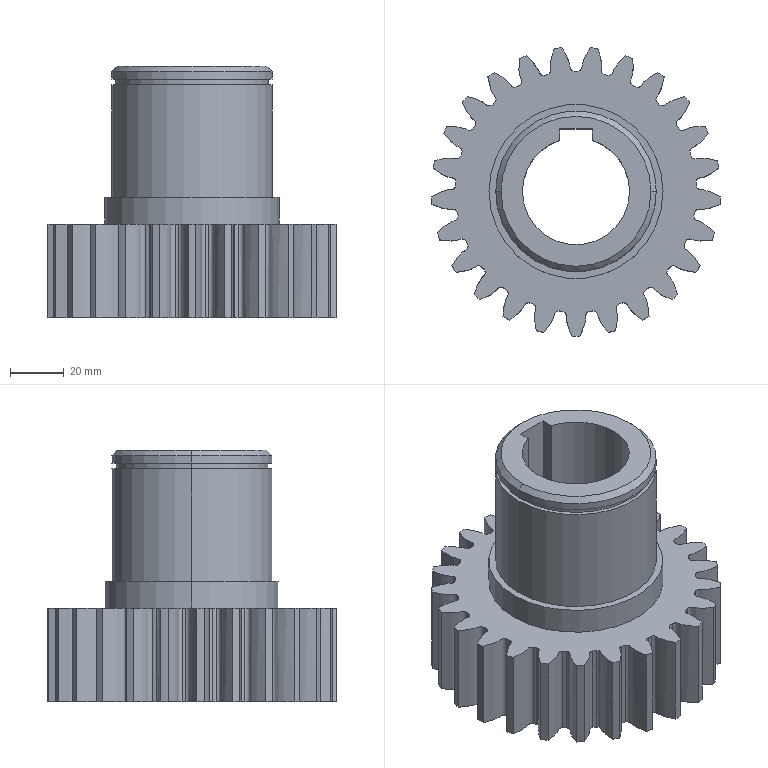Component | SolidWorks | DriveGearPart-1 | 1 solid | 122 faces | volume 318720 mm3 | cylinder 61 | spline 50 | plane 9 | cone 2 | commonest cylinder face diameters 108 x25 90 x25 60 x4 40 x3 57 x2 65 x2